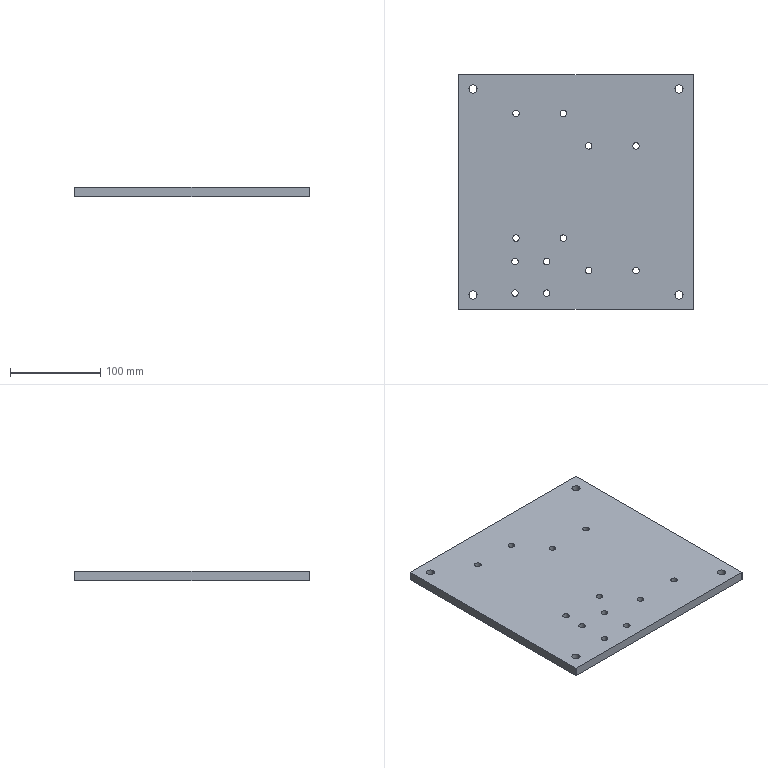CAM job | Mastercam | mm | 5 operations | part box 260 x 260 x 10
1. Facing | 24 - 100 平铣刀
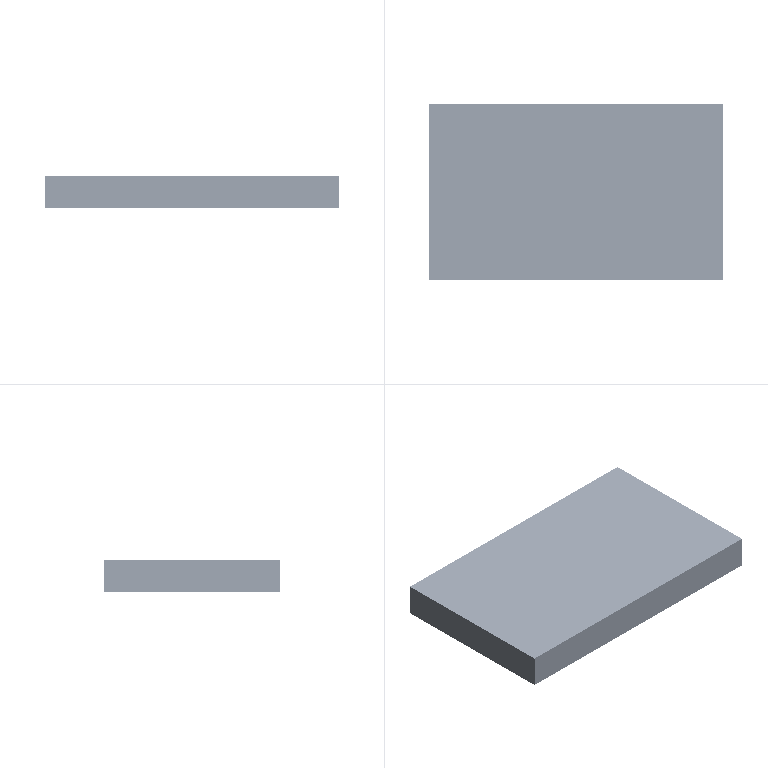2. Contour (Ramp) | 9 - 10 平铣刀
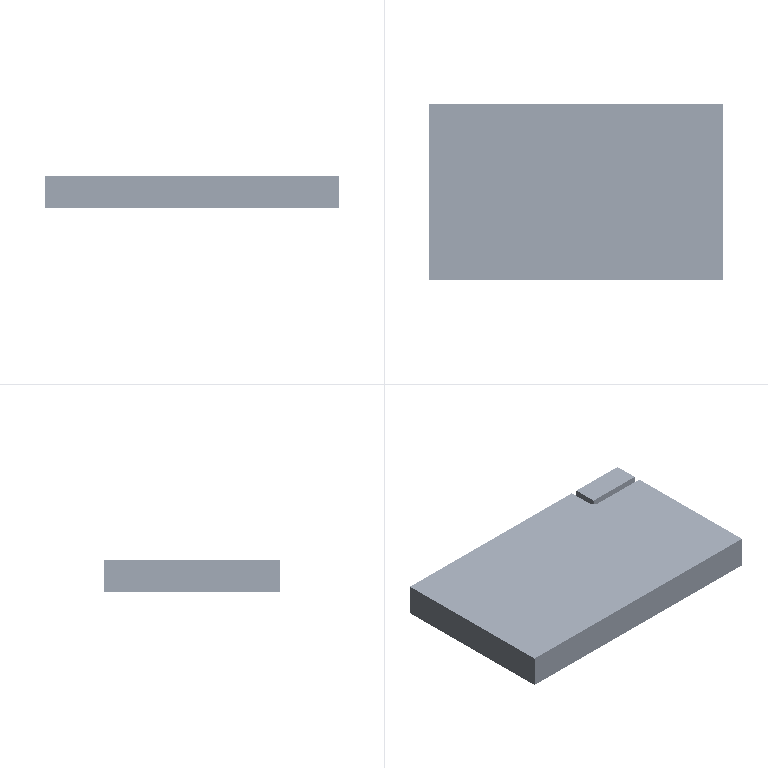3. Contour (2D) | 10 - 10 平铣刀
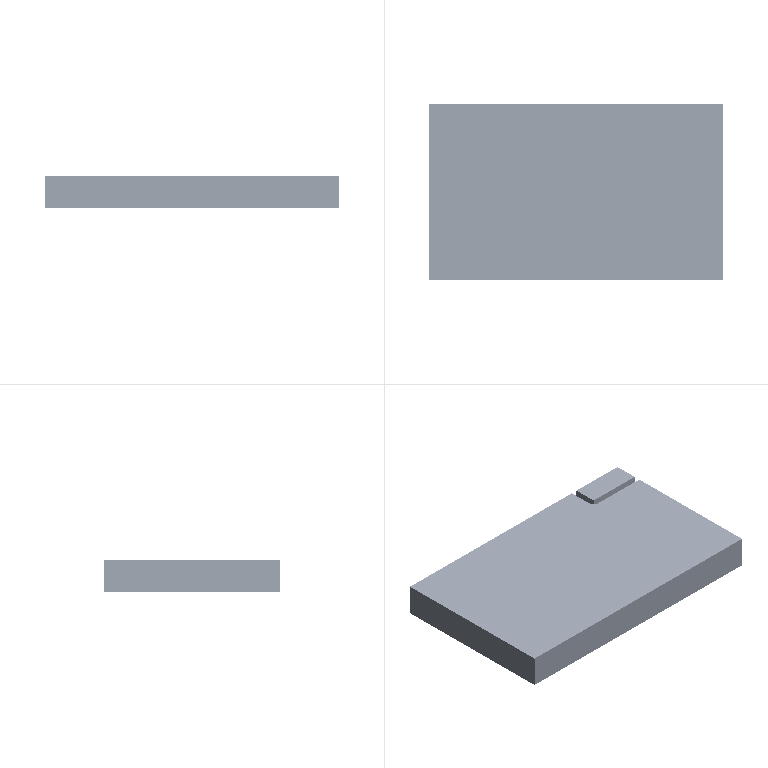4. Drill/Counterbore | 7 - 6 倒角刀
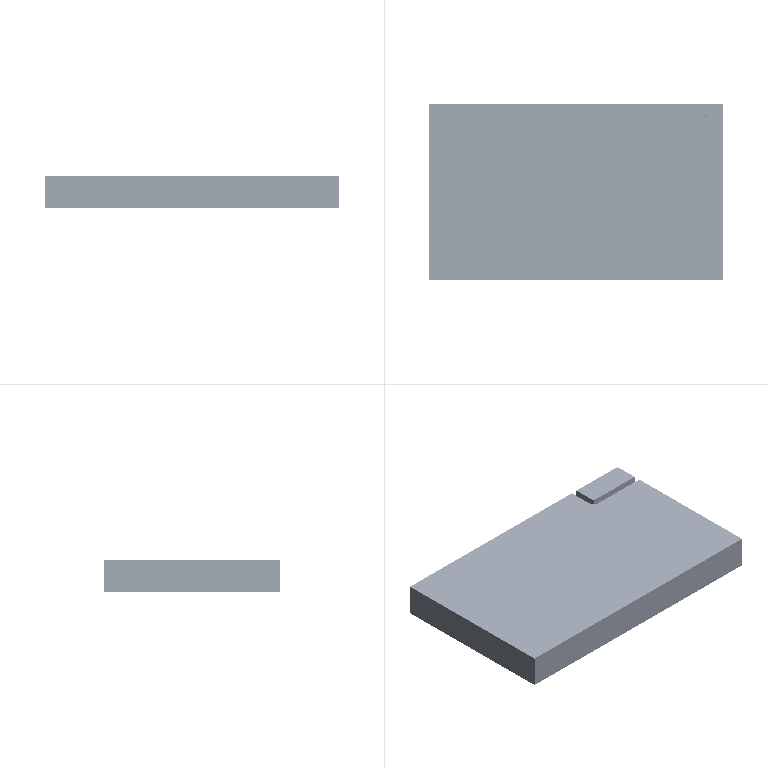5. Contour (2D chamfer) | 7 - 6 倒角刀